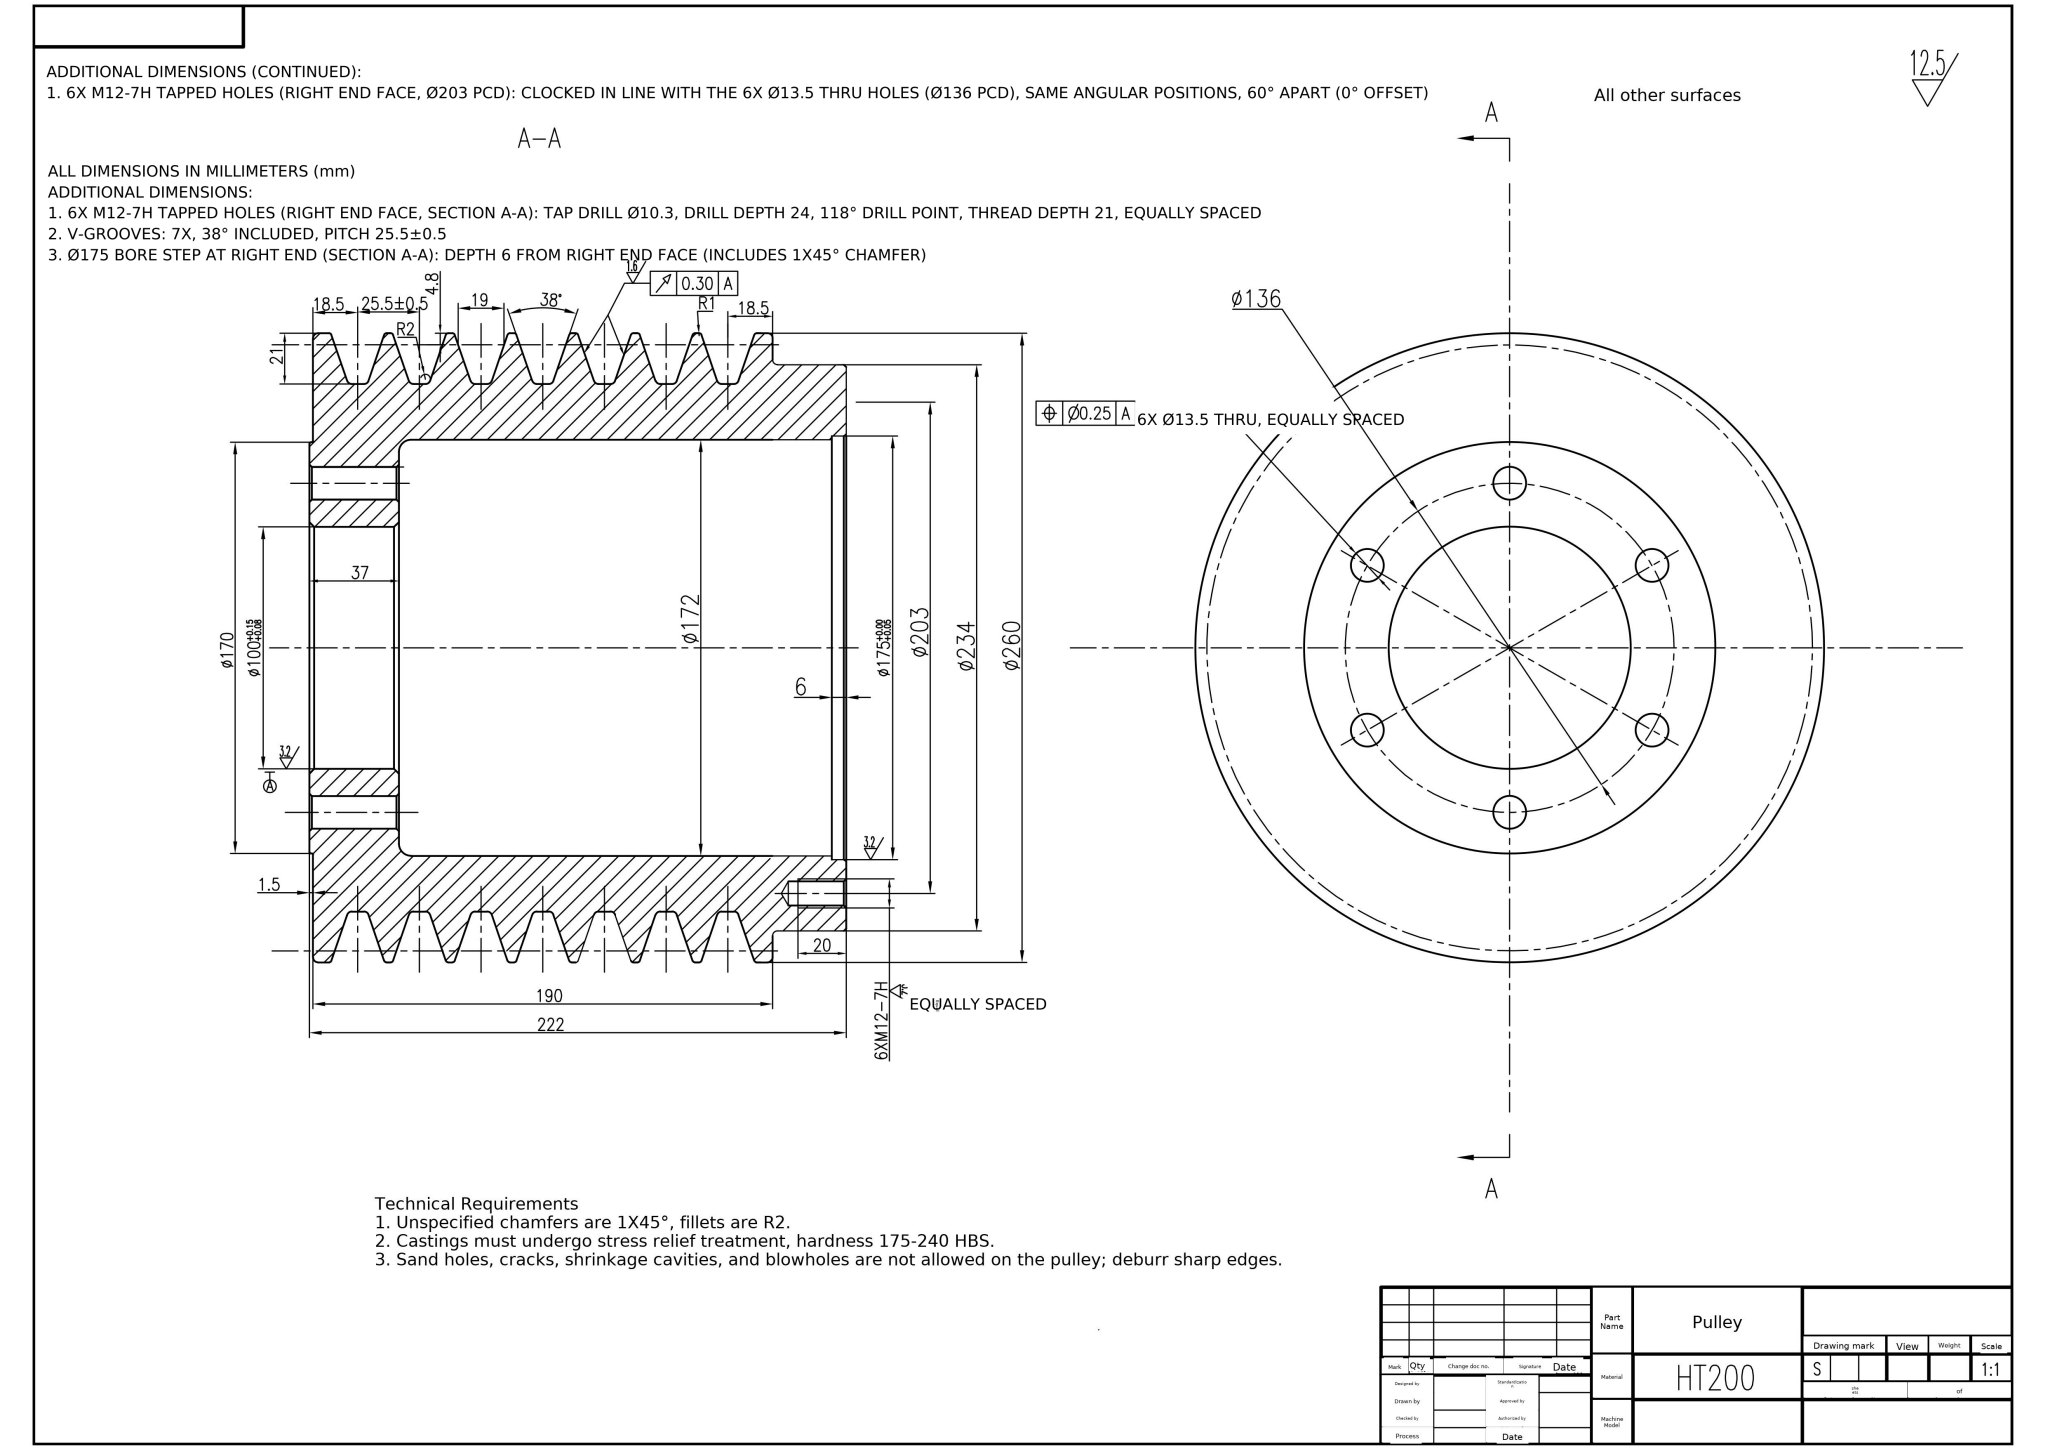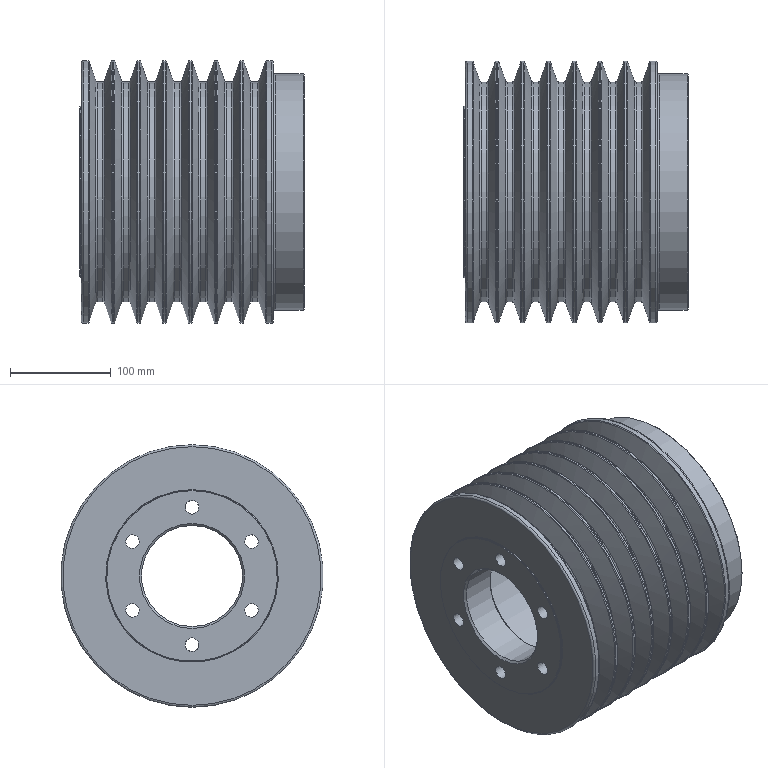Part | NX | mm | 1 solid | 102 faces | box 222 x 260 x 260 mm | volume 5110435 mm3 | torus 33 | cylinder 32 | cone 31 | plane 6 | commonest cylinder face diameters 260 x8 218 x7 13.5 x6 10.3 x6 234 x1 175 x1 172 x1 100 x1